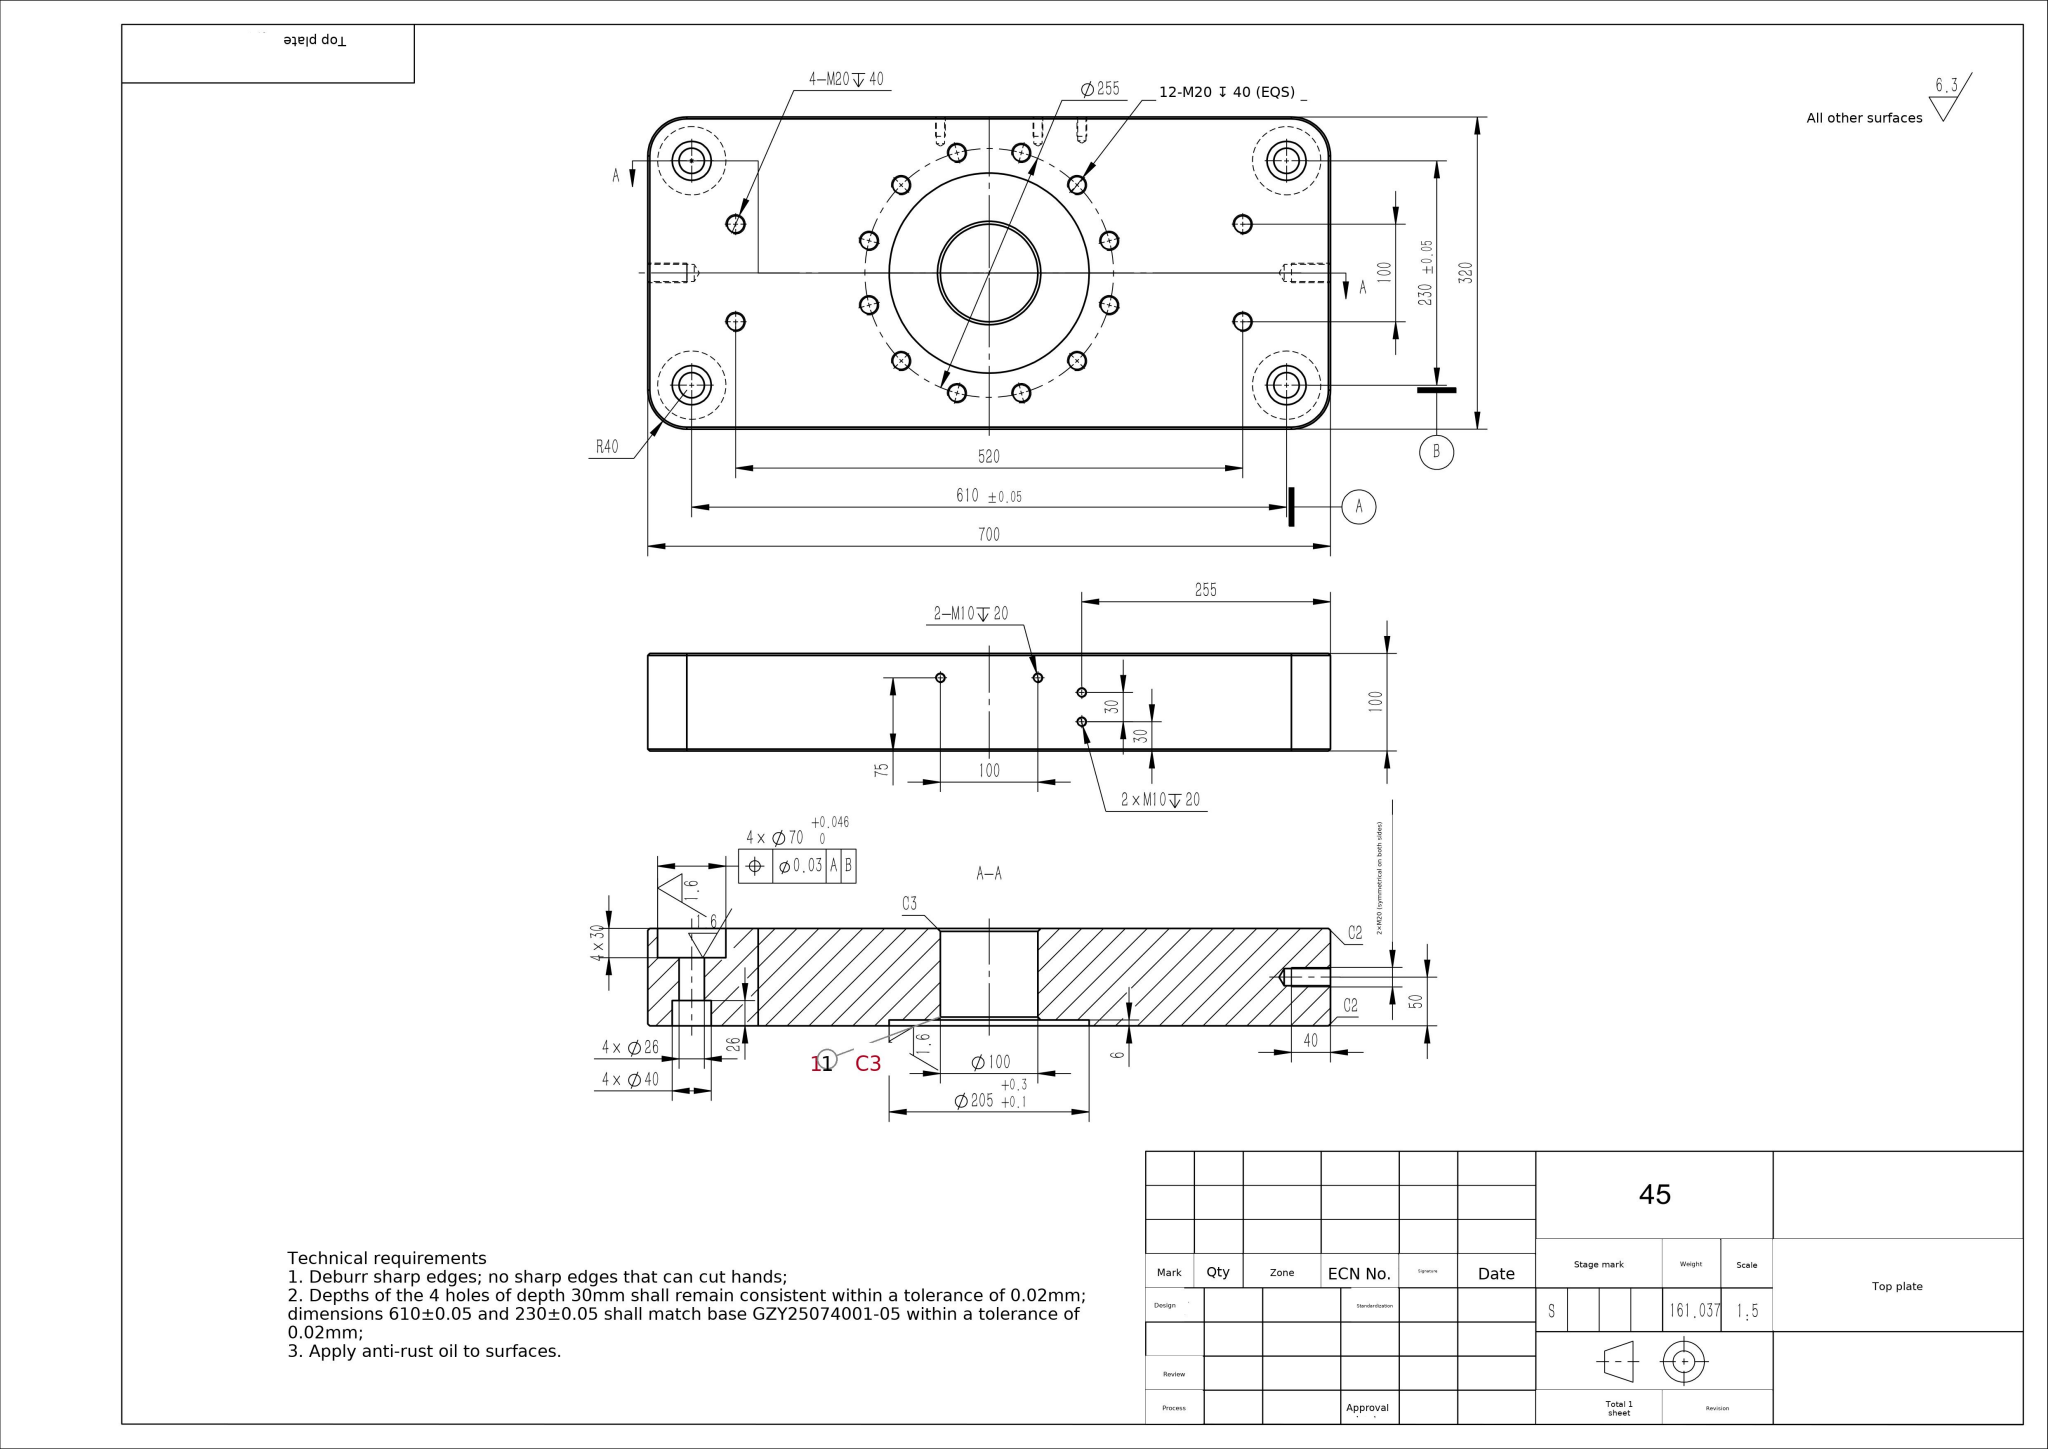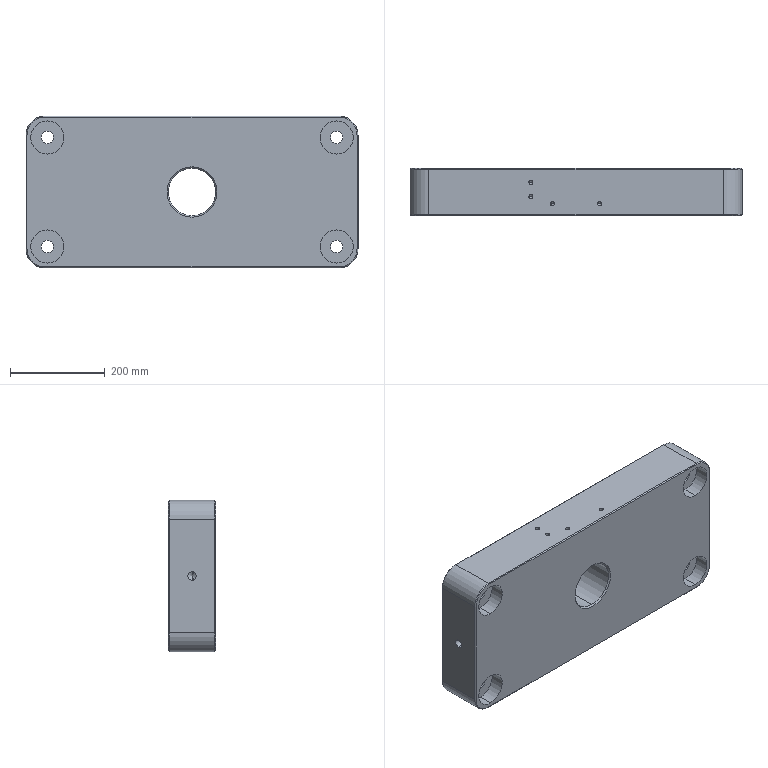Part | SolidWorks | mm | material 45 | 1 solid | 155 faces | box 700 x 100 x 320 mm | volume 20388320 mm3 | cylinder 76 | cone 56 | plane 23 | commonest cylinder face diameters 17.5 x36 8.5 x8 26 x8 40 x8 70 x8 80 x4 205 x2 100 x2
build123d program:
from build123d import *

# Parameters (mm, degrees)
BOSS_EXTRUDE1_DEPTH    = 100
CUT_EXTRUDE1_START     = -100
SKETCH3_R              = 35
CUT_EXTRUDE1_DEPTH     = 30
CUT_EXTRUDE6_START     = -100
SKETCH5_R              = 20
CUT_EXTRUDE6_DEPTH     = 26
SKETCH26_R             = 13
CUT_EXTRUDE7_DEPTH     = 398.618
SKETCH6_R              = 50
CUT_EXTRUDE4_DEPTH     = 398.618
CUT_EXTRUDE5_START     = -100
SKETCH7_R              = 102.5
CUT_EXTRUDE5_DEPTH     = 6
CHAMFER1_SIZE          = 3
CIRPATTERN1_COUNT      = 12
M10_TAPPED_HOLE2_D     = 8.5
M10_TAPPED_HOLE2_DEPTH = 27.5
M10_TAPPED_HOLE2_TIP   = 2.554
CHAMFER2_SIZE          = 2


with BuildPart() as part:
    # Sketch2 → Boss-Extrude1 (new body)
    with BuildSketch(Plane(origin=(0, 0, 0), x_dir=(1, 0, 0), z_dir=(0, 1, 0))):
        with BuildLine():
            Line((-310, 160), (310, 160))
            ThreePointArc((310, 160), (338.284, 148.284), (350, 120))
            Line((350, 120), (350, -120))
            ThreePointArc((350, -120), (338.284, -148.284), (310, -160))
            Line((310, -160), (-310, -160))
            ThreePointArc((-310, -160), (-338.284, -148.284), (-350, -120))
            Line((-350, -120), (-350, 120))
            ThreePointArc((-350, 120), (-338.284, 148.284), (-310, 160))
        make_face()
    extrude(amount=-BOSS_EXTRUDE1_DEPTH)

    # Sketch3 → Cut-Extrude1 (cut)
    with BuildSketch(Plane(origin=(0, 0, 0), x_dir=(1, 0, 0), z_dir=(0, 1, 0)).offset(CUT_EXTRUDE1_START)):
        with Locations(Location((-305, 115, 0), (0, 0, 270))):
            Circle(SKETCH3_R)
        with Locations(Location((305, 115, 0), (0, 0, 90))):
            Circle(SKETCH3_R)
        with Locations(Location((305, -115, 0), (0, 0, 270))):
            Circle(SKETCH3_R)
        with Locations(Location((-305, -115, 0), (0, 0, 90))):
            Circle(SKETCH3_R)
    extrude(amount=CUT_EXTRUDE1_DEPTH, mode=Mode.SUBTRACT)

    # Sketch5 → Cut-Extrude6 (cut)
    with BuildSketch(Plane.XZ.offset(100).offset(CUT_EXTRUDE6_START)):
        with Locations(Location((-305, 115, 0), (0, 0, 90))):
            Circle(SKETCH5_R)
        with Locations(Location((-305, -115, 0), (0, 0, 90))):
            Circle(SKETCH5_R)
        with Locations(Location((305, 115, 0), (0, 0, 90))):
            Circle(SKETCH5_R)
        with Locations(Location((305, -115, 0), (0, 0, 90))):
            Circle(SKETCH5_R)
    extrude(amount=CUT_EXTRUDE6_DEPTH, mode=Mode.SUBTRACT)

    # Sketch26 → Cut-Extrude7 (cut, through all)
    with BuildSketch(Plane.XZ.offset(100)):
        with Locations(Location((-305, 115, 0), (0, 0, 270))):
            Circle(SKETCH26_R)
        with Locations(Location((305, 115, 0), (0, 0, 270))):
            Circle(SKETCH26_R)
        with Locations(Location((305, -115, 0), (0, 0, 270))):
            Circle(SKETCH26_R)
        with Locations(Location((-305, -115, 0), (0, 0, 270))):
            Circle(SKETCH26_R)
    extrude(amount=-CUT_EXTRUDE7_DEPTH, mode=Mode.SUBTRACT)

    # Sketch6 → Cut-Extrude4 (cut, through all)
    with BuildSketch(Plane(origin=(0, 0, 0), x_dir=(1, 0, 0), z_dir=(0, 1, 0))):
        with Locations(Location((0, 0, 0), (0, 0, 270))):
            Circle(SKETCH6_R)
    extrude(amount=-CUT_EXTRUDE4_DEPTH, mode=Mode.SUBTRACT)

    # Sketch7 → Cut-Extrude5 (cut)
    with BuildSketch(Plane.XZ.offset(100).offset(CUT_EXTRUDE5_START)):
        with Locations(Location((0, 0, 0), (0, 0, 270))):
            Circle(SKETCH7_R)
    extrude(amount=CUT_EXTRUDE5_DEPTH, mode=Mode.SUBTRACT)

    # Chamfer1
    chamfer1_edges = [part.edges().sort_by_distance(p)[0] for p in [
        (0, -100, -50),
        (0, -6, -50),
    ]]
    chamfer(chamfer1_edges, length=CHAMFER1_SIZE)

    # Sketch25 → M20 Tapped Hole4 (revolve, cut)
    with BuildSketch(Plane(origin=(32.999, 0, -123.156), x_dir=(0, 0, 1), z_dir=(1, 0, 0))):
        Polygon((0, 0), (0, 57.758), (8.75, 52.5), (8.75, 0), align=None)
    m20_tapped_hole4 = revolve(axis=Axis((32.999, 6.35, -123.156), (0, -1, 0)), mode=Mode.SUBTRACT)

    # CirPattern1: M20 Tapped Hole4 ×12 about axis
    cirpattern1_axis = Axis((0, 0, 0), (0, 1, 0))
    for i in range(1, CIRPATTERN1_COUNT):
        add(m20_tapped_hole4.rotate(cirpattern1_axis, i * 360 / CIRPATTERN1_COUNT), mode=Mode.SUBTRACT)

    # Sketch11 → M20 Tapped Hole2 (revolve, cut)
    with BuildSketch(Plane(origin=(260, 0, -50), x_dir=(0, 0, 1), z_dir=(1, 0, 0))):
        Polygon((0, 0), (0, 57.758), (8.75, 52.5), (8.75, 0), align=None)
    m20_tapped_hole2 = revolve(axis=Axis((260, 6.35, -50), (0, -1, 0)), mode=Mode.SUBTRACT)

    # Mirror1: M20 Tapped Hole2 across plane
    add(m20_tapped_hole2.mirror(Plane(origin=(0, 0, 0), x_dir=(0, 0, 1), z_dir=(1, 0, 0))), mode=Mode.SUBTRACT)

    # Mirror1 at the second plane: M20 Tapped Hole2 across plane
    add(m20_tapped_hole2.mirror(Plane.XY), mode=Mode.SUBTRACT)

    # Mirror1 at the second plane copy 1 sketc → Mirror1 at the second plane copy 1 (revolve, cut)
    with BuildSketch(Plane(origin=(-260, 0, 50), x_dir=(0, 0, -1), z_dir=(-1, 0, 0))):
        Polygon((0, 0), (0, 57.758), (8.75, 52.5), (8.75, 0), align=None)
    revolve(axis=Axis((-260, 6.35, 50), (0, -1, 0)), mode=Mode.SUBTRACT)

    # M10 Tapped Hole2
    with Locations(Plane(origin=(-95, -60, 160), x_dir=(1, 0, 0), z_dir=(0, 0, 1))):
        with Locations((0, 0), (0, 30)):
            Hole(M10_TAPPED_HOLE2_D / 2, depth=M10_TAPPED_HOLE2_DEPTH)
            with Locations((0, 0, -(M10_TAPPED_HOLE2_DEPTH + M10_TAPPED_HOLE2_TIP / 2))):  # 118° drill point
                Cone(0, M10_TAPPED_HOLE2_D / 2, M10_TAPPED_HOLE2_TIP, mode=Mode.SUBTRACT)

    # Sketch19 → M10 Tapped Hole3 (revolve, cut)
    with BuildSketch(Plane(origin=(50, -75, 160), x_dir=(0, -1, 0), z_dir=(1, 0, 0))):
        Polygon((0, 0), (0, 30.054), (4.25, 27.5), (4.25, 0), align=None)
    m10_tapped_hole3 = revolve(axis=Axis((50, -75, 166.35), (0, 0, -1)), mode=Mode.SUBTRACT)

    # Mirror3: M10 Tapped Hole3 across plane
    add(m10_tapped_hole3.mirror(Plane(origin=(0, 0, 0), x_dir=(0, 0, 1), z_dir=(1, 0, 0))), mode=Mode.SUBTRACT)

    # Chamfer2
    chamfer2_edges = [part.edges().sort_by_distance(p)[0] for p in [
        (0, 0, -160),
        (338.284, 0, -148.284),
        (350, 0, 0),
        (338.284, 0, 148.284),
        (338.284, -100, -148.284),
        (0, -100, -160),
        (-338.284, -100, -148.284),
        (-350, -100, 0),
        (-338.284, -100, 148.284),
        (0, -100, 160),
        (338.284, -100, 148.284),
        (0, 0, 160),
        (350, -100, 0),
        (-338.284, 0, 148.284),
        (-350, 0, 0),
        (-338.284, 0, -148.284),
    ]]
    chamfer(chamfer2_edges, length=CHAMFER2_SIZE)

    # Sketch22 → M20 Tapped Hole3 (revolve, cut)
    with BuildSketch(Plane(origin=(350, -50.04, 0), x_dir=(0, 0, -1), z_dir=(0, 1, 0))):
        Polygon((0, 0), (0, 57.758), (8.75, 52.5), (8.75, 0), align=None)
    m20_tapped_hole3 = revolve(axis=Axis((356.35, -50.04, 0), (-1, 0, 0)), mode=Mode.SUBTRACT)

    # Mirror4: M20 Tapped Hole3 across plane
    add(m20_tapped_hole3.mirror(Plane(origin=(0, 0, 0), x_dir=(0, 0, 1), z_dir=(1, 0, 0))), mode=Mode.SUBTRACT)


solid = part.part